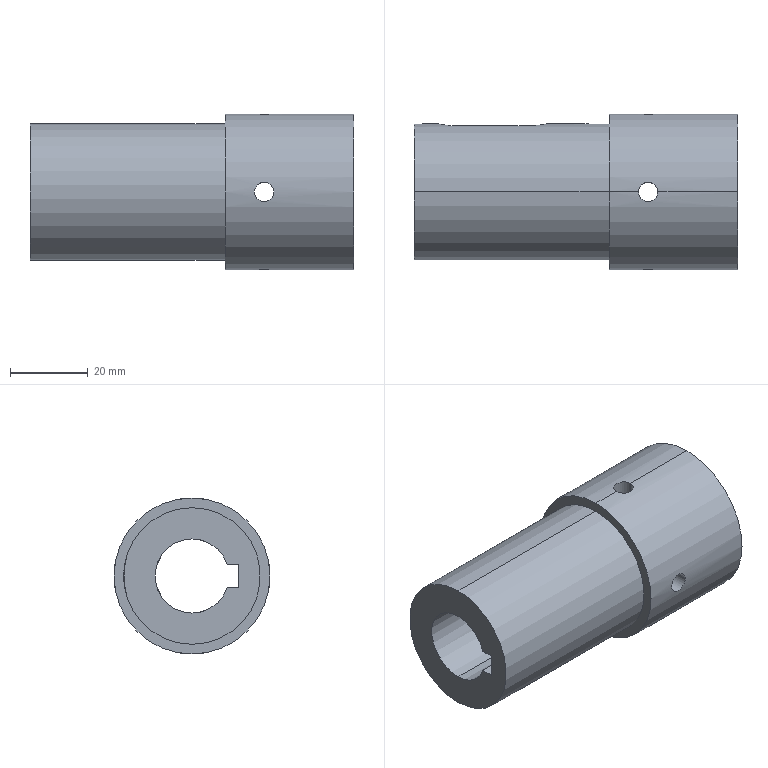Component | SolidWorks | ElectricalBoxAssembly2-1_MotorShaftSleeve-1 | 1 solid | 27 faces | box 83 x 40 x 40 mm | volume 63122 mm3 | cylinder 18 | plane 9 | commonest cylinder face diameters 5 x8 8 x3 19 x3 40 x2 35 x2
build123d program:
from build123d import *

# Parameters (mm, degrees)
SKETCH1_R           = 17.5
BOSS_EXTRUDE1_DEPTH = 83
SKETCH3_R           = 9.5
CUT_EXTRUDE1_DEPTH  = 87.611
SKETCH4_W           = 6
SKETCH4_H           = 3
CUT_EXTRUDE2_DEPTH  = 87.611
CUT_EXTRUDE3_DEPTH  = 4
SKETCH6_R           = 20
SKETCH6_R_2         = 15
BOSS_EXTRUDE2_DEPTH = 33
SKETCH9_W           = 2.5
SKETCH9_H           = 37.5
CIRPATTERN1_COUNT   = 4


with BuildPart() as part:
    # Sketch1 → Boss-Extrude1 (new body)
    with BuildSketch(Plane.XY):
        Circle(SKETCH1_R)
    extrude(amount=BOSS_EXTRUDE1_DEPTH)

    # Sketch3 → Cut-Extrude1 (cut, through all)
    with BuildSketch(Plane(origin=(0, 0, 0), x_dir=(-1, 0, 0), z_dir=(0, 0, -1))):
        Circle(SKETCH3_R)
    extrude(amount=-CUT_EXTRUDE1_DEPTH, mode=Mode.SUBTRACT)

    # Sketch4 → Cut-Extrude2 (cut, through all)
    with BuildSketch(Plane(origin=(0, 0, 0), x_dir=(-1, 0, 0), z_dir=(0, 0, -1))):
        with Locations((0, 10.514)):
            Rectangle(SKETCH4_W, SKETCH4_H)
    extrude(amount=-CUT_EXTRUDE2_DEPTH, mode=Mode.SUBTRACT)

    # Sketch5 → Cut-Extrude3 (cut)
    with BuildSketch(Plane(origin=(0, -17.5, 0), x_dir=(1, 0, 0), z_dir=(0, 1, 0))):
        with BuildLine():
            Line((-4, -73), (-4, -53))
            ThreePointArc((-4, -53), (0, -49), (4, -53))
            Line((4, -53), (4, -73))
            ThreePointArc((4, -73), (0, -77), (-4, -73))
        make_face()
    extrude(amount=CUT_EXTRUDE3_DEPTH, mode=Mode.SUBTRACT)

    # Sketch6 → Boss-Extrude2 (add)
    with BuildSketch(Plane.XY.offset(33)):
        Circle(SKETCH6_R)
        Circle(SKETCH6_R_2, mode=Mode.SUBTRACT)
    extrude(amount=-BOSS_EXTRUDE2_DEPTH)

    # Sketch9 → M6 Tapped Hole1 (revolve, cut)
    with BuildSketch(Plane(origin=(0, 17.5, 23), x_dir=(0, 0, 1), z_dir=(1, 0, 0))):
        with Locations((1.25, 18.75)):
            Rectangle(SKETCH9_W, SKETCH9_H)
    m6_tapped_hole1 = revolve(axis=Axis((0, 23.85, 23), (0, -1, 0)), mode=Mode.SUBTRACT)

    # CirPattern1: M6 Tapped Hole1 ×4 about axis
    cirpattern1_axis = Axis((0, 0, 83), (0, 0, -1))
    for i in range(1, CIRPATTERN1_COUNT):
        add(m6_tapped_hole1.rotate(cirpattern1_axis, i * 360 / CIRPATTERN1_COUNT), mode=Mode.SUBTRACT)


solid = part.part

# Placed as in the assembly
solid = solid.moved(Location((761.968, 214.666, 1526.399), (180, -90, 0)))